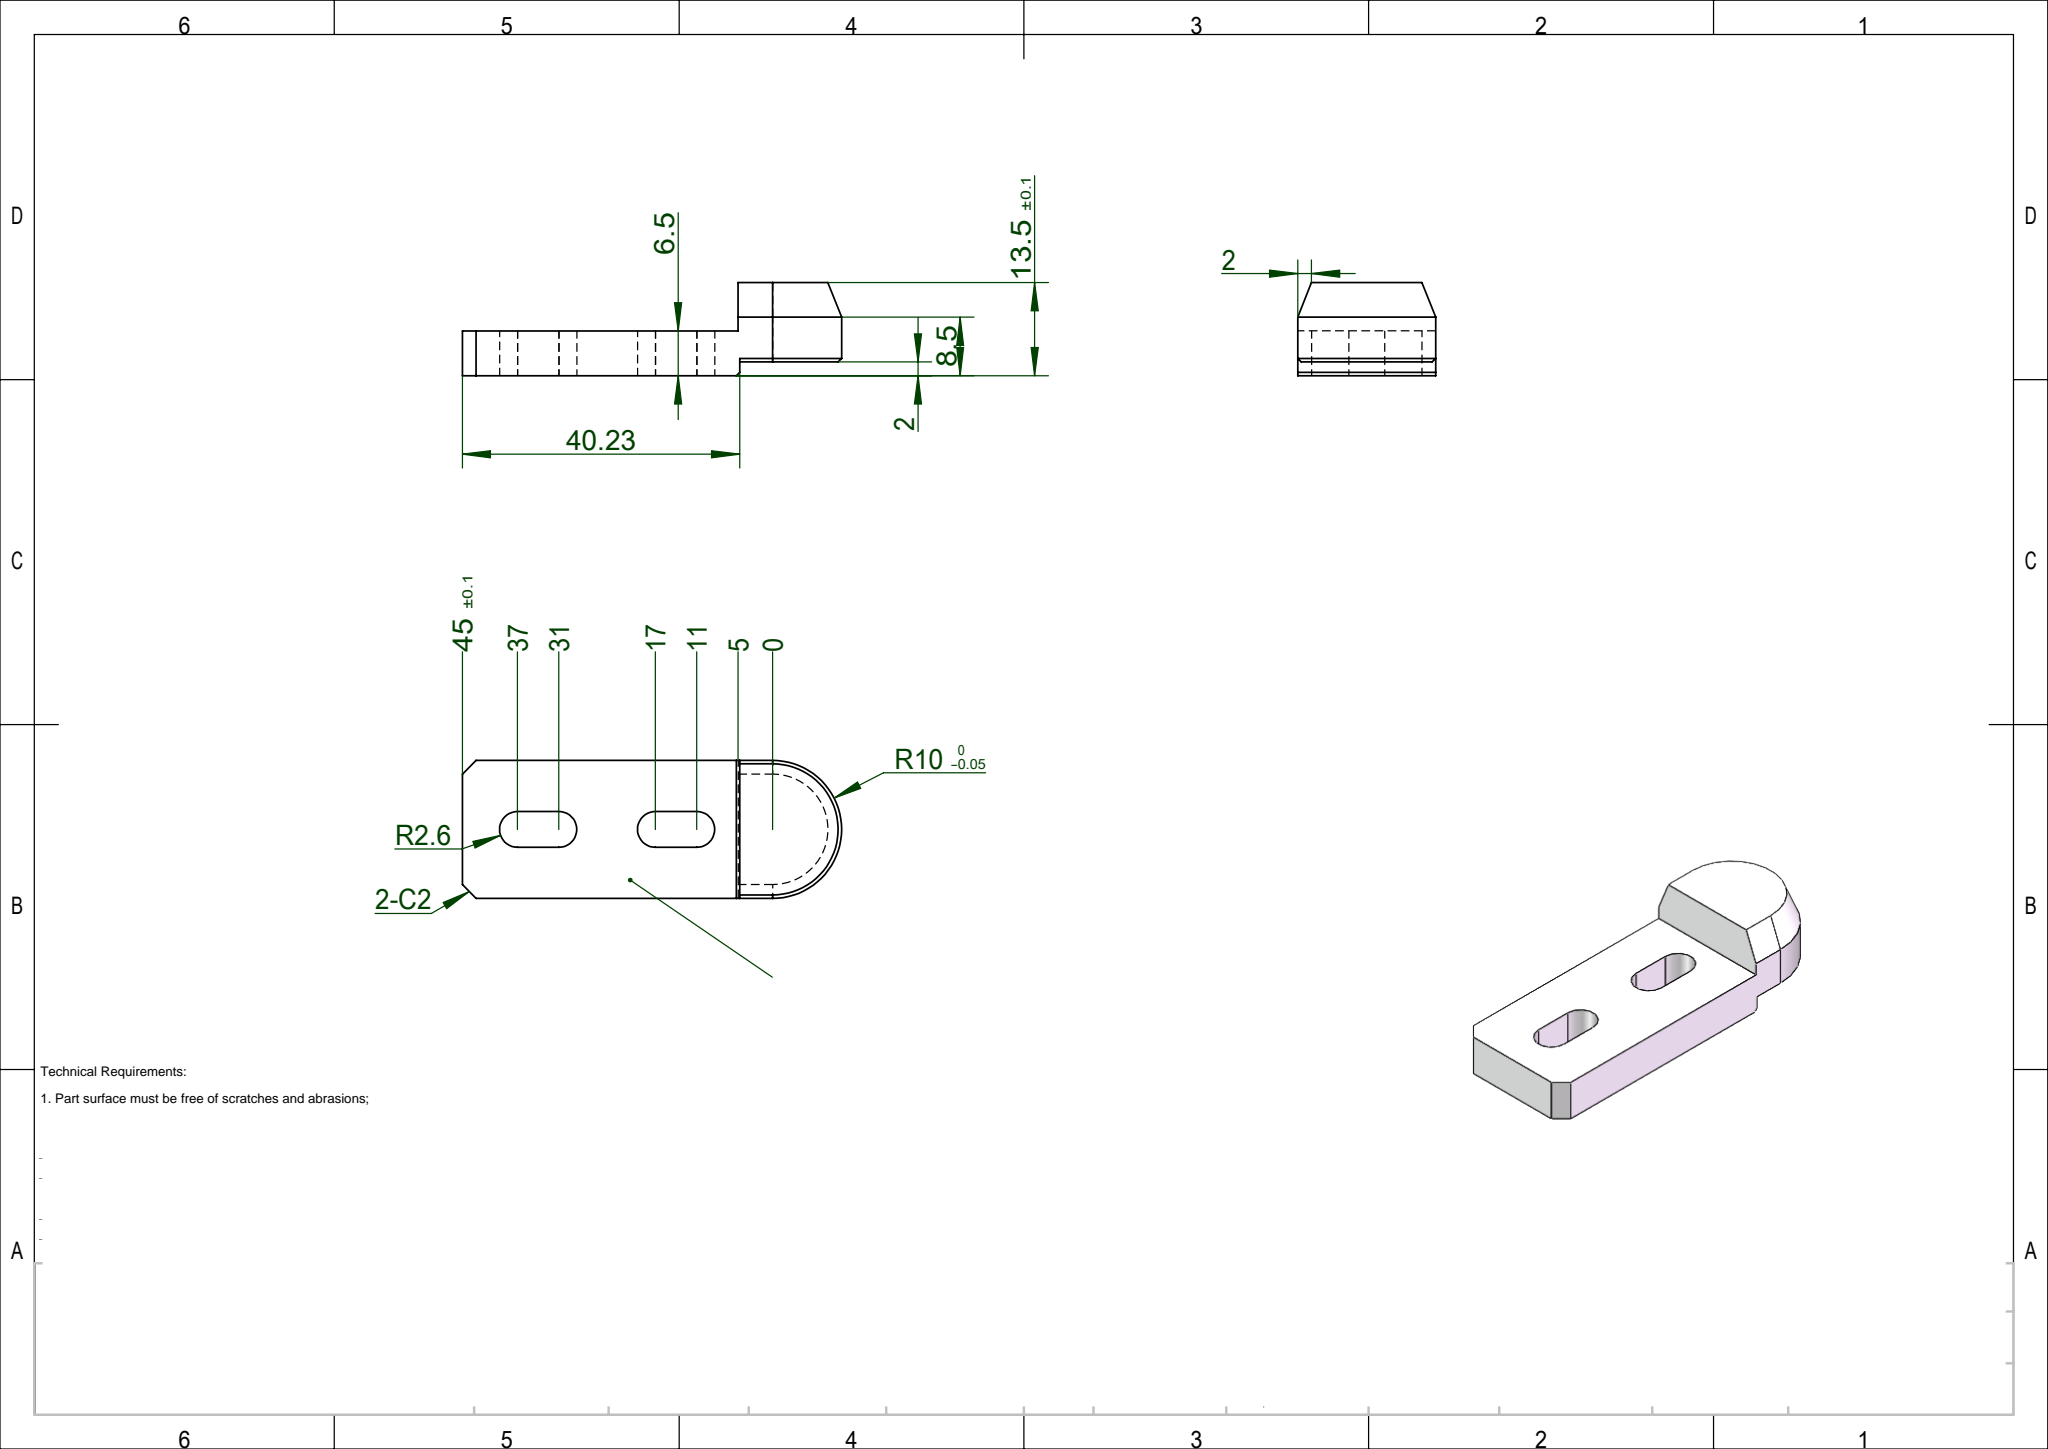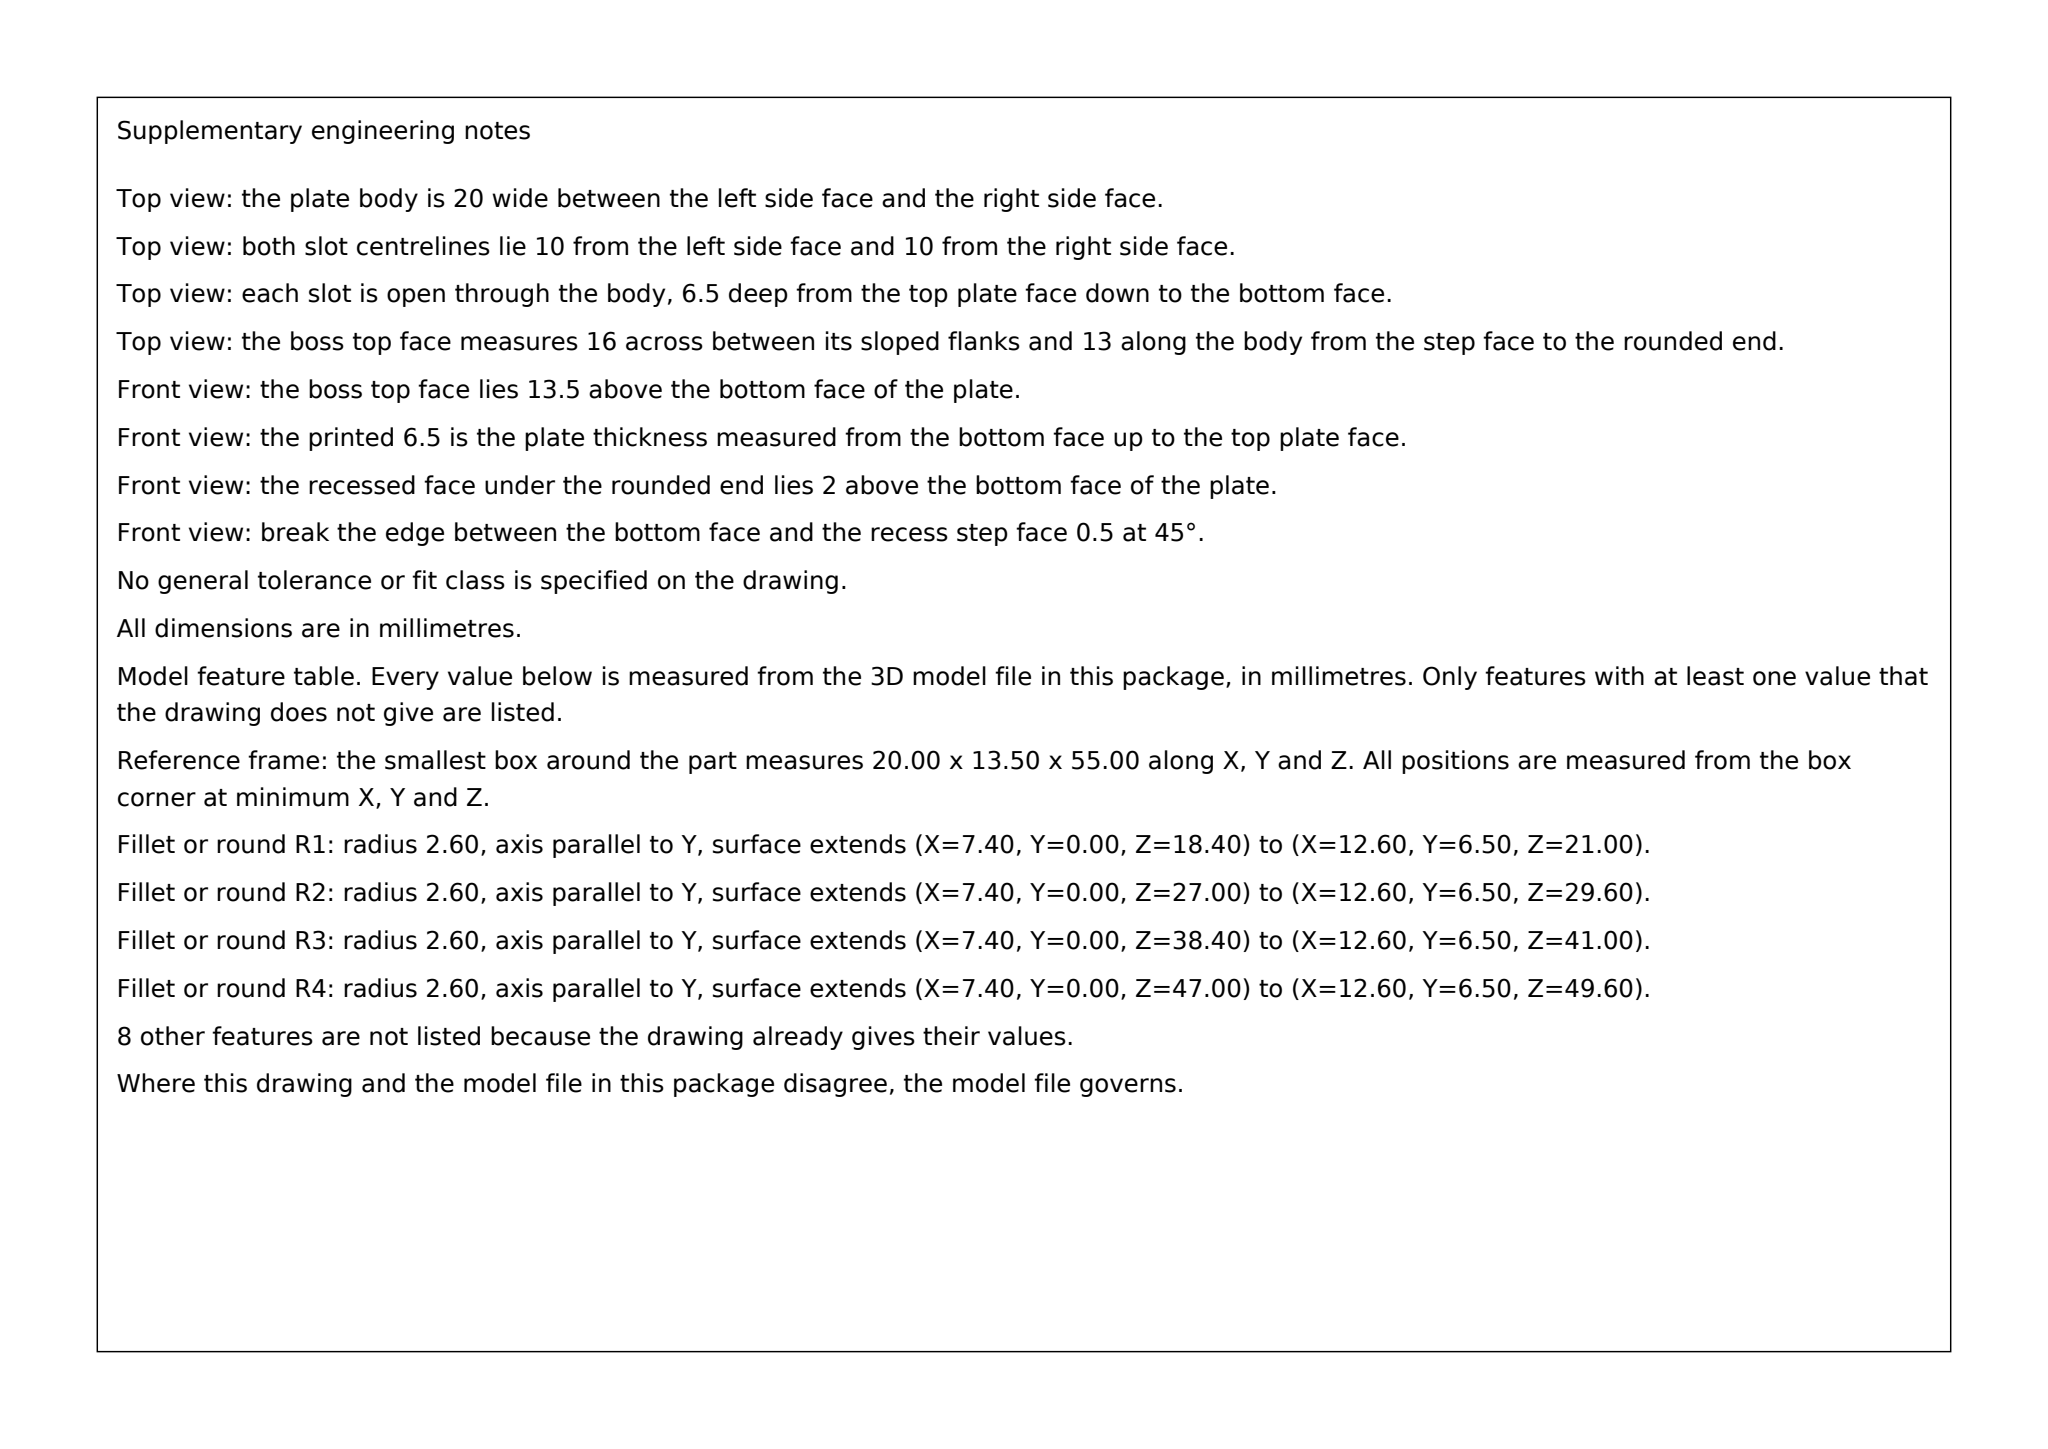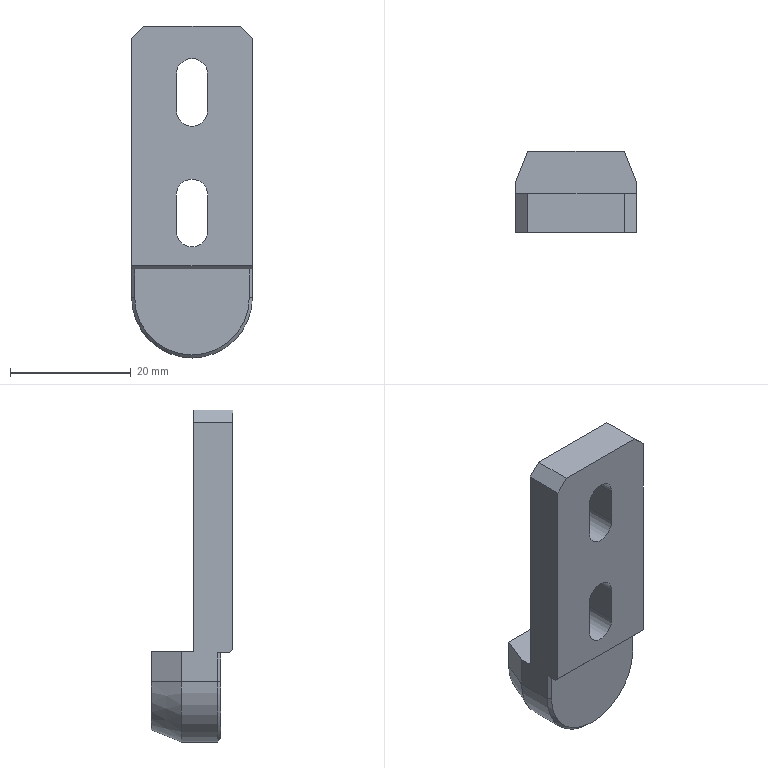Part | SolidWorks | mm | 1 solid | 31 faces | box 20 x 13.5 x 55 mm | volume 7254 mm3 | plane 20 | cylinder 8 | cone 3 | commonest cylinder face diameters 5.2 x6 20 x2
Drawing notes:
OVERALL WIDTH 20, R10 END ARC TANG BOTH SIDES | from the solid: bbox_xyz X=20; dia20 cyl axis y at x=10 => tangent to x=0 and x=20 planes
2 SLOTS SYM ABT CL, SLOT AXES 10 FROM EA SIDE | from the solid: all 5.2 dia slot-end cyls at x=10.0, bbox X=20 => on centreline
BOSS TOP: 43.6° INCL CONE REF Ø16, 2 PL; 90° INCL CONE REF Ø19 | from the solid: cones[included_angle,ref_dia]: [43.6,16.0]x2 and [90.0,19.0]x1
BOSS FULL WIDTH 20, SLOPE FACES SYM ABT CL | from the solid: x axis_planes at 0.0 and 20.0 bound boss; cones coaxial on x=10 CL
2 BTM RELIEF AT R10 END EXTENDS 15 FROM END FACE | from the solid: y planes 0 and 2 (2 deep); z plane at 15.0, round-end arc centre z=10 R10 => end at z=0
build123d program:
from build123d import *
from OCP.BRepFilletAPI import BRepFilletAPI_MakeChamfer

# Parameters (mm, degrees)
BOSS_EXTRUDE1_DEPTH = 13.5
SKETCH2_W           = 49.69
SKETCH2_H           = 11.405
CUT_EXTRUDE1_DEPTH  = 111
CUT_EXTRUDE2_DEPTH  = 111
CHAMFER1_SIZE       = 5
CHAMFER1_SIZE2      = 2
CHAMFER2_SIZE       = 2
SKETCH4_W           = 31.068
SKETCH4_H           = 15
CUT_EXTRUDE3_DEPTH  = 2
CHAMFER3_SIZE       = 0.5


with BuildPart() as part:
    # Sketch1 → Boss-Extrude1 (new body)
    with BuildSketch(Plane(origin=(0, 0, 0), x_dir=(1, 0, 0), z_dir=(0, 1, 0))):
        with BuildLine():
            Line((-10, -45), (10, -45))
            Line((10, -45), (10, 0))
            ThreePointArc((10, 0), (0, 10), (-10, 0))
            Line((-10, 0), (-10, -45))
        make_face()
    extrude(amount=BOSS_EXTRUDE1_DEPTH)

    # Sketch2 → Cut-Extrude1 (cut)
    with BuildSketch(Plane(origin=(10, 0, 0), x_dir=(0, 0, -1), z_dir=(1, 0, 0))):
        with Locations((-29.845, 12.202)):
            Rectangle(SKETCH2_W, SKETCH2_H)
    extrude(amount=-CUT_EXTRUDE1_DEPTH, mode=Mode.SUBTRACT)

    # Sketch3 → Cut-Extrude2 (cut)
    with BuildSketch(Plane(origin=(0, 6.5, 0), x_dir=(1, 0, 0), z_dir=(0, 1, 0))):
        with BuildLine():
            Line((-2.6, -17), (-2.6, -11))
            ThreePointArc((-2.6, -11), (0, -8.4), (2.6, -11))
            Line((2.6, -11), (2.6, -17))
            ThreePointArc((2.6, -17), (0, -19.6), (-2.6, -17))
        make_face()
        with BuildLine():
            Line((-2.6, -37), (-2.6, -31))
            ThreePointArc((-2.6, -31), (0, -28.4), (2.6, -31))
            Line((2.6, -31), (2.6, -37))
            ThreePointArc((2.6, -37), (0, -39.6), (-2.6, -37))
        make_face()
    extrude(amount=-CUT_EXTRUDE2_DEPTH, mode=Mode.SUBTRACT)

    # Chamfer1: one chamfer whose edges measure the first distance from different faces: ONE call of the kernel's chamfer builder (chamfer() names one face for all edges)
    chamfer1_edges_1 = [part.edges().sort_by_distance(p)[0] for p in [
        (0, 13.5, -10),
    ]]
    chamfer1_side_1 = [part.faces().sort_by_distance(p)[0] for p in [
        (0, 6.75, -10),
    ]]
    chamfer1_edges_2 = [part.edges().sort_by_distance(p)[0] for p in [
        (10, 13.5, 2.5),
    ]]
    chamfer1_side_2 = [part.faces().sort_by_distance(p)[0] for p in [
        (10, 3.971, 20.363),
    ]]
    chamfer1_edges_3 = [part.edges().sort_by_distance(p)[0] for p in [
        (-10, 13.5, 2.5),
    ]]
    chamfer1_side_3 = [part.faces().sort_by_distance(p)[0] for p in [
        (-10, 3.971, 20.363),
    ]]
    chamfer1 = BRepFilletAPI_MakeChamfer(part.part.solid().wrapped)
    for e in chamfer1_edges_1:
        chamfer1.Add(CHAMFER1_SIZE, CHAMFER1_SIZE2, e.wrapped, chamfer1_side_1[0].wrapped)  # the first distance lies on this face
    for e in chamfer1_edges_2:
        chamfer1.Add(CHAMFER1_SIZE, CHAMFER1_SIZE2, e.wrapped, chamfer1_side_2[0].wrapped)  # the first distance lies on this face
    for e in chamfer1_edges_3:
        chamfer1.Add(CHAMFER1_SIZE, CHAMFER1_SIZE2, e.wrapped, chamfer1_side_3[0].wrapped)  # the first distance lies on this face
    add(Compound.cast(chamfer1.Shape()), mode=Mode.REPLACE)

    # Chamfer2
    chamfer2_edges = [part.edges().sort_by_distance(p)[0] for p in [
        (10, 3.25, 45),
        (-10, 3.25, 45),
    ]]
    chamfer(chamfer2_edges, length=CHAMFER2_SIZE)

    # Sketch4 → Cut-Extrude3 (cut)
    with BuildSketch(Plane.XZ):
        with Locations((0.3331, -2.728)):
            Rectangle(SKETCH4_W, SKETCH4_H)
    extrude(amount=-CUT_EXTRUDE3_DEPTH, mode=Mode.SUBTRACT)

    # Chamfer3
    chamfer3_edges = [part.edges().sort_by_distance(p)[0] for p in [
        (0, 0, 4.772),
        (0, 2, -10),
        (-10, 2, 2.386),
        (10, 2, 2.386),
    ]]
    chamfer(chamfer3_edges, length=CHAMFER3_SIZE)


solid = part.part